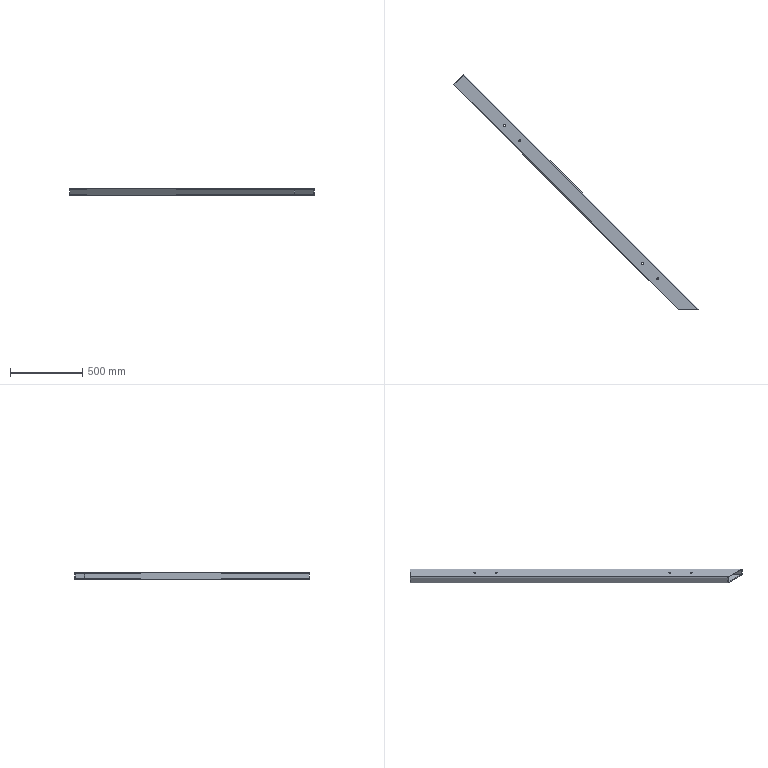Component | NX | INCL_SUPP_FRAME_CONN_BEAM | 1 solid | 26 faces | volume 2551753 mm3 | cylinder 16 | plane 10 | commonest cylinder face diameters 8 x8 13 x8